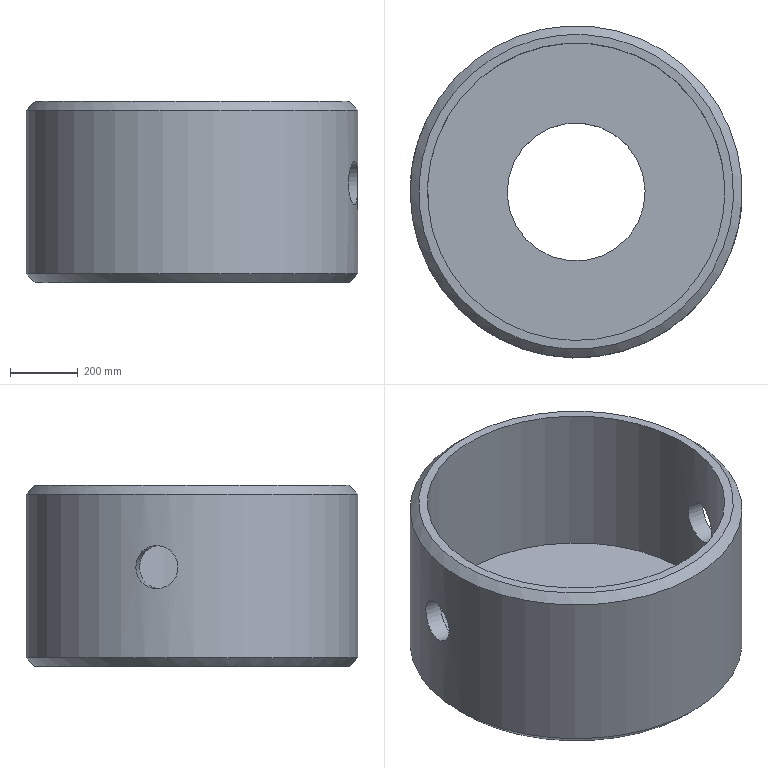Component | NX | 10 | 1 solid | 10 faces | volume 111762553 mm3 | cylinder 5 | plane 3 | cone 2 | commonest cylinder face diameters 127 x2 977.9 x1 876.3 x1 406.4 x1